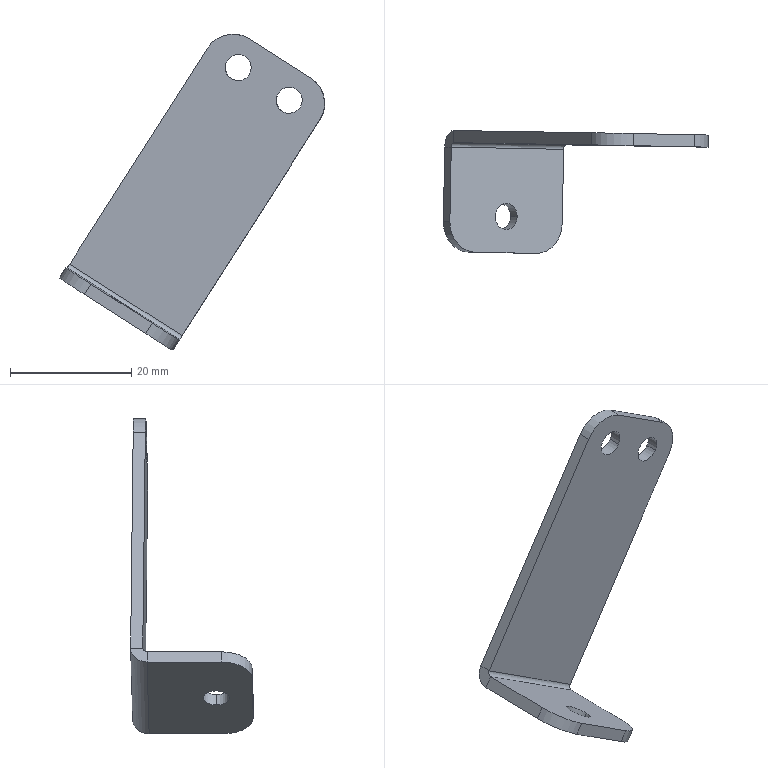Component | SolidWorks | DM17A08-02-003-1 | 1 solid | 24 faces | box 43.81 x 20.26 x 52.08 mm | volume 2829 mm3 | cylinder 12 | plane 12 | commonest cylinder face diameters 4.3 x6 10 x4 5.473 x1 1.473 x1
STEP:
#1=CARTESIAN_POINT('',(24.753,18.88,37.793));
#2=VERTEX_POINT('',#1);
#3=CARTESIAN_POINT('',(24.895,18.877,37.702));
#4=VERTEX_POINT('',#3);
#5=CARTESIAN_POINT('',(24.824,18.878,37.747));
#6=DIRECTION('',(-0.01873,-0.9998,0.));
#7=DIRECTION('',(0.843,-0.01579,-0.5377));
#8=AXIS2_PLACEMENT_3D('',#5,#6,#7);
#9=CIRCLE('',#8,0.08465);
#10=EDGE_CURVE('',#2,#4,#9,.T.);
#11=ORIENTED_EDGE('',*,*,#10,.F.);
#12=CARTESIAN_POINT('',(24.751,18.801,37.793));
#13=VERTEX_POINT('',#12);
#14=CARTESIAN_POINT('',(24.751,18.801,37.793));
#15=DIRECTION('',(-0.01873,-0.9998,0.));
#16=VECTOR('',#15,39.37);
#17=LINE('',#14,#16);
#18=EDGE_CURVE('',#2,#13,#17,.T.);
#19=ORIENTED_EDGE('',*,*,#18,.T.);
#20=CARTESIAN_POINT('',(24.894,18.798,37.702));
#21=VERTEX_POINT('',#20);
#22=CARTESIAN_POINT('',(24.823,18.8,37.747));
#23=DIRECTION('',(-0.01873,-0.9998,0.));
#24=DIRECTION('',(0.843,-0.01579,-0.5377));
#25=AXIS2_PLACEMENT_3D('',#22,#23,#24);
#26=CIRCLE('',#25,0.08465);
#27=EDGE_CURVE('',#13,#21,#26,.T.);
#28=ORIENTED_EDGE('',*,*,#27,.T.);
#29=CARTESIAN_POINT('',(24.894,18.798,37.702));
#30=DIRECTION('',(-0.01873,-0.9998,0.));
#31=VECTOR('',#30,39.37);
#32=LINE('',#29,#31);
#33=EDGE_CURVE('',#4,#21,#32,.T.);
#34=ORIENTED_EDGE('',*,*,#33,.F.);
#35=EDGE_LOOP('',(#11,#19,#28,#34));
#36=FACE_OUTER_BOUND('',#35,.T.);
#37=CARTESIAN_POINT('',(24.823,18.8,37.747));
#38=DIRECTION('',(-0.01873,-0.9998,0.));
#39=DIRECTION('',(0.843,-0.01579,-0.5377));
#40=AXIS2_PLACEMENT_3D('',#37,#38,#39);
#41=CYLINDRICAL_SURFACE('',#40,0.08465);
#42=ADVANCED_FACE('',(#36),#41,.F.);
#43=CARTESIAN_POINT('',(24.421,18.886,38.005));
#44=VERTEX_POINT('',#43);
#45=CARTESIAN_POINT('',(24.563,18.883,37.914));
#46=VERTEX_POINT('',#45);
#47=CARTESIAN_POINT('',(24.492,18.885,37.959));
#48=DIRECTION('',(-0.01873,-0.9998,0.));
#49=DIRECTION('',(0.843,-0.01579,-0.5377));
#50=AXIS2_PLACEMENT_3D('',#47,#48,#49);
#51=CIRCLE('',#50,0.08465);
#52=EDGE_CURVE('',#44,#46,#51,.T.);
#53=ORIENTED_EDGE('',*,*,#52,.F.);
#54=CARTESIAN_POINT('',(24.419,18.807,38.005));
#55=VERTEX_POINT('',#54);
#56=CARTESIAN_POINT('',(24.419,18.807,38.005));
#57=DIRECTION('',(-0.01873,-0.9998,0.));
#58=VECTOR('',#57,39.37);
#59=LINE('',#56,#58);
#60=EDGE_CURVE('',#44,#55,#59,.T.);
#61=ORIENTED_EDGE('',*,*,#60,.T.);
#62=CARTESIAN_POINT('',(24.562,18.805,37.914));
#63=VERTEX_POINT('',#62);
#64=CARTESIAN_POINT('',(24.491,18.806,37.959));
#65=DIRECTION('',(-0.01873,-0.9998,0.));
#66=DIRECTION('',(0.843,-0.01579,-0.5377));
#67=AXIS2_PLACEMENT_3D('',#64,#65,#66);
#68=CIRCLE('',#67,0.08465);
#69=EDGE_CURVE('',#55,#63,#68,.T.);
#70=ORIENTED_EDGE('',*,*,#69,.T.);
#71=CARTESIAN_POINT('',(24.562,18.805,37.914));
#72=DIRECTION('',(-0.01873,-0.9998,0.));
#73=VECTOR('',#72,39.37);
#74=LINE('',#71,#73);
#75=EDGE_CURVE('',#46,#63,#74,.T.);
#76=ORIENTED_EDGE('',*,*,#75,.F.);
#77=EDGE_LOOP('',(#53,#61,#70,#76));
#78=FACE_OUTER_BOUND('',#77,.T.);
#79=CARTESIAN_POINT('',(24.491,18.806,37.959));
#80=DIRECTION('',(-0.01873,-0.9998,0.));
#81=DIRECTION('',(0.843,-0.01579,-0.5377));
#82=AXIS2_PLACEMENT_3D('',#79,#80,#81);
#83=CYLINDRICAL_SURFACE('',#82,0.08465);
#84=ADVANCED_FACE('',(#78),#83,.F.);
#85=CARTESIAN_POINT('',(23.809,18.346,36.38));
#86=VERTEX_POINT('',#85);
#87=CARTESIAN_POINT('',(23.666,18.349,36.471));
#88=VERTEX_POINT('',#87);
#89=CARTESIAN_POINT('',(23.738,18.347,36.426));
#90=DIRECTION('',(-0.5377,0.01007,-0.8431));
#91=DIRECTION('',(0.01873,0.9998,0.));
#92=AXIS2_PLACEMENT_3D('',#89,#90,#91);
#93=CIRCLE('',#92,0.08465);
#94=EDGE_CURVE('',#86,#88,#93,.T.);
#95=ORIENTED_EDGE('',*,*,#94,.F.);
#96=CARTESIAN_POINT('',(23.767,18.347,36.314));
#97=VERTEX_POINT('',#96);
#98=CARTESIAN_POINT('',(23.767,18.347,36.314));
#99=DIRECTION('',(-0.5377,0.01007,-0.8431));
#100=VECTOR('',#99,39.37);
#101=LINE('',#98,#100);
#102=EDGE_CURVE('',#86,#97,#101,.T.);
#103=ORIENTED_EDGE('',*,*,#102,.T.);
#104=CARTESIAN_POINT('',(23.624,18.35,36.405));
#105=VERTEX_POINT('',#104);
#106=CARTESIAN_POINT('',(23.695,18.348,36.36));
#107=DIRECTION('',(-0.5377,0.01007,-0.8431));
#108=DIRECTION('',(-0.843,0.01579,0.5377));
#109=AXIS2_PLACEMENT_3D('',#106,#107,#108);
#110=CIRCLE('',#109,0.08465);
#111=EDGE_CURVE('',#97,#105,#110,.T.);
#112=ORIENTED_EDGE('',*,*,#111,.T.);
#113=CARTESIAN_POINT('',(23.624,18.35,36.405));
#114=DIRECTION('',(-0.5377,0.01007,-0.8431));
#115=VECTOR('',#114,39.37);
#116=LINE('',#113,#115);
#117=EDGE_CURVE('',#88,#105,#116,.T.);
#118=ORIENTED_EDGE('',*,*,#117,.F.);
#119=EDGE_LOOP('',(#95,#103,#112,#118));
#120=FACE_OUTER_BOUND('',#119,.T.);
#121=CARTESIAN_POINT('',(23.695,18.348,36.36));
#122=DIRECTION('',(-0.5377,0.01007,-0.8431));
#123=DIRECTION('',(-0.843,0.01579,0.5377));
#124=AXIS2_PLACEMENT_3D('',#121,#122,#123);
#125=CYLINDRICAL_SURFACE('',#124,0.08465);
#126=ADVANCED_FACE('',(#120),#125,.F.);
#127=CARTESIAN_POINT('',(24.069,18.785,36.127));
#128=VERTEX_POINT('',#127);
#129=CARTESIAN_POINT('',(24.111,18.784,36.193));
#130=VERTEX_POINT('',#129);
#131=CARTESIAN_POINT('',(24.069,18.785,36.127));
#132=DIRECTION('',(0.5377,-0.01007,0.8431));
#133=VECTOR('',#132,39.37);
#134=LINE('',#131,#133);
#135=EDGE_CURVE('',#128,#130,#134,.T.);
#136=ORIENTED_EDGE('',*,*,#135,.F.);
#137=CARTESIAN_POINT('',(24.129,18.891,36.217));
#138=VERTEX_POINT('',#137);
#139=CARTESIAN_POINT('',(24.126,18.784,36.217));
#140=DIRECTION('',(-0.843,0.01579,0.5377));
#141=DIRECTION('',(0.01873,0.9998,0.));
#142=AXIS2_PLACEMENT_3D('',#139,#140,#141);
#143=CIRCLE('',#142,0.1077);
#144=EDGE_CURVE('',#138,#128,#143,.T.);
#145=ORIENTED_EDGE('',*,*,#144,.F.);
#146=CARTESIAN_POINT('',(24.127,18.813,36.217));
#147=VERTEX_POINT('',#146);
#148=CARTESIAN_POINT('',(24.127,18.813,36.217));
#149=DIRECTION('',(0.01873,0.9998,-0.));
#150=VECTOR('',#149,39.37);
#151=LINE('',#148,#150);
#152=EDGE_CURVE('',#147,#138,#151,.T.);
#153=ORIENTED_EDGE('',*,*,#152,.F.);
#154=CARTESIAN_POINT('',(24.126,18.784,36.217));
#155=DIRECTION('',(-0.843,0.01579,0.5377));
#156=DIRECTION('',(0.01873,0.9998,0.));
#157=AXIS2_PLACEMENT_3D('',#154,#155,#156);
#158=CIRCLE('',#157,0.029);
#159=EDGE_CURVE('',#147,#130,#158,.T.);
#160=ORIENTED_EDGE('',*,*,#159,.T.);
#161=EDGE_LOOP('',(#136,#145,#153,#160));
#162=FACE_OUTER_BOUND('',#161,.T.);
#163=CARTESIAN_POINT('',(24.069,18.785,36.127));
#164=DIRECTION('',(0.843,-0.01579,-0.5377));
#165=DIRECTION('',(0.01873,0.9998,-0.));
#166=AXIS2_PLACEMENT_3D('',#163,#164,#165);
#167=PLANE('',#166);
#168=ADVANCED_FACE('',(#162),#167,.T.);
#169=CARTESIAN_POINT('',(24.102,18.301,36.193));
#170=VERTEX_POINT('',#169);
#171=CARTESIAN_POINT('',(24.113,18.892,36.193));
#172=DIRECTION('',(-0.01873,-0.9998,0.));
#173=VECTOR('',#172,39.37);
#174=LINE('',#171,#173);
#175=EDGE_CURVE('',#130,#170,#174,.T.);
#176=ORIENTED_EDGE('',*,*,#175,.T.);
#177=CARTESIAN_POINT('',(24.06,18.302,36.127));
#178=VERTEX_POINT('',#177);
#179=CARTESIAN_POINT('',(24.117,18.301,36.217));
#180=DIRECTION('',(-0.5377,0.01007,-0.8431));
#181=VECTOR('',#180,39.37);
#182=LINE('',#179,#181);
#183=EDGE_CURVE('',#170,#178,#182,.T.);
#184=ORIENTED_EDGE('',*,*,#183,.T.);
#185=CARTESIAN_POINT('',(24.071,18.892,36.127));
#186=DIRECTION('',(-0.01873,-0.9998,0.));
#187=VECTOR('',#186,39.37);
#188=LINE('',#185,#187);
#189=EDGE_CURVE('',#128,#178,#188,.T.);
#190=ORIENTED_EDGE('',*,*,#189,.F.);
#191=ORIENTED_EDGE('',*,*,#135,.T.);
#192=EDGE_LOOP('',(#176,#184,#190,#191));
#193=FACE_OUTER_BOUND('',#192,.T.);
#194=CARTESIAN_POINT('',(24.127,18.813,36.217));
#195=DIRECTION('',(0.843,-0.01579,-0.5377));
#196=DIRECTION('',(0.01873,0.9998,-0.));
#197=AXIS2_PLACEMENT_3D('',#194,#195,#196);
#198=PLANE('',#197);
#199=ADVANCED_FACE('',(#193),#198,.T.);
#200=CARTESIAN_POINT('',(23.398,18.905,36.683));
#201=VERTEX_POINT('',#200);
#202=CARTESIAN_POINT('',(23.397,18.826,36.683));
#203=VERTEX_POINT('',#202);
#204=CARTESIAN_POINT('',(23.398,18.905,36.683));
#205=DIRECTION('',(-0.01873,-0.9998,0.));
#206=VECTOR('',#205,39.37);
#207=LINE('',#204,#206);
#208=EDGE_CURVE('',#201,#203,#207,.T.);
#209=ORIENTED_EDGE('',*,*,#208,.F.);
#210=CARTESIAN_POINT('',(23.338,18.798,36.592));
#211=VERTEX_POINT('',#210);
#212=CARTESIAN_POINT('',(23.396,18.797,36.683));
#213=DIRECTION('',(-0.843,0.01579,0.5377));
#214=DIRECTION('',(0.01873,0.9998,0.));
#215=AXIS2_PLACEMENT_3D('',#212,#213,#214);
#216=CIRCLE('',#215,0.1077);
#217=EDGE_CURVE('',#201,#211,#216,.T.);
#218=ORIENTED_EDGE('',*,*,#217,.T.);
#219=CARTESIAN_POINT('',(23.381,18.798,36.659));
#220=VERTEX_POINT('',#219);
#221=CARTESIAN_POINT('',(23.381,18.798,36.659));
#222=DIRECTION('',(-0.5377,0.01007,-0.8431));
#223=VECTOR('',#222,39.37);
#224=LINE('',#221,#223);
#225=EDGE_CURVE('',#220,#211,#224,.T.);
#226=ORIENTED_EDGE('',*,*,#225,.F.);
#227=CARTESIAN_POINT('',(23.396,18.797,36.683));
#228=DIRECTION('',(-0.843,0.01579,0.5377));
#229=DIRECTION('',(0.01873,0.9998,0.));
#230=AXIS2_PLACEMENT_3D('',#227,#228,#229);
#231=CIRCLE('',#230,0.029);
#232=EDGE_CURVE('',#203,#220,#231,.T.);
#233=ORIENTED_EDGE('',*,*,#232,.F.);
#234=EDGE_LOOP('',(#209,#218,#226,#233));
#235=FACE_OUTER_BOUND('',#234,.T.);
#236=CARTESIAN_POINT('',(23.398,18.905,36.683));
#237=DIRECTION('',(-0.843,0.01579,0.5377));
#238=DIRECTION('',(-0.01873,-0.9998,0.));
#239=AXIS2_PLACEMENT_3D('',#236,#237,#238);
#240=PLANE('',#239);
#241=ADVANCED_FACE('',(#235),#240,.T.);
#242=CARTESIAN_POINT('',(24.292,18.81,38.086));
#243=VERTEX_POINT('',#242);
#244=CARTESIAN_POINT('',(24.397,18.808,38.252));
#245=DIRECTION('',(-0.5377,0.01007,-0.8431));
#246=VECTOR('',#245,39.37);
#247=LINE('',#244,#246);
#248=EDGE_CURVE('',#243,#203,#247,.T.);
#249=ORIENTED_EDGE('',*,*,#248,.F.);
#250=CARTESIAN_POINT('',(24.293,18.888,38.086));
#251=VERTEX_POINT('',#250);
#252=CARTESIAN_POINT('',(24.291,18.781,38.086));
#253=DIRECTION('',(0.01873,0.9998,-0.));
#254=VECTOR('',#253,39.37);
#255=LINE('',#252,#254);
#256=EDGE_CURVE('',#243,#251,#255,.T.);
#257=ORIENTED_EDGE('',*,*,#256,.T.);
#258=CARTESIAN_POINT('',(24.399,18.886,38.252));
#259=DIRECTION('',(-0.5377,0.01007,-0.8431));
#260=VECTOR('',#259,39.37);
#261=LINE('',#258,#260);
#262=EDGE_CURVE('',#251,#201,#261,.T.);
#263=ORIENTED_EDGE('',*,*,#262,.T.);
#264=ORIENTED_EDGE('',*,*,#208,.T.);
#265=EDGE_LOOP('',(#249,#257,#263,#264));
#266=FACE_OUTER_BOUND('',#265,.T.);
#267=CARTESIAN_POINT('',(23.381,18.798,36.659));
#268=DIRECTION('',(-0.843,0.01579,0.5377));
#269=DIRECTION('',(-0.01873,-0.9998,0.));
#270=AXIS2_PLACEMENT_3D('',#267,#268,#269);
#271=PLANE('',#270);
#272=ADVANCED_FACE('',(#266),#271,.T.);
#273=CARTESIAN_POINT('',(23.738,18.347,36.426));
#274=DIRECTION('',(-0.5377,0.01007,-0.8431));
#275=DIRECTION('',(0.01873,0.9998,0.));
#276=AXIS2_PLACEMENT_3D('',#273,#274,#275);
#277=CIRCLE('',#276,0.08465);
#278=EDGE_CURVE('',#88,#86,#277,.T.);
#279=ORIENTED_EDGE('',*,*,#278,.T.);
#280=ORIENTED_EDGE('',*,*,#94,.T.);
#281=EDGE_LOOP('',(#279,#280));
#282=FACE_BOUND('',#281,.T.);
#283=CARTESIAN_POINT('',(23.932,18.108,36.299));
#284=VERTEX_POINT('',#283);
#285=CARTESIAN_POINT('',(23.534,18.115,36.553));
#286=VERTEX_POINT('',#285);
#287=CARTESIAN_POINT('',(24.098,18.104,36.193));
#288=DIRECTION('',(-0.843,0.01579,0.5377));
#289=VECTOR('',#288,39.37);
#290=LINE('',#287,#289);
#291=EDGE_CURVE('',#284,#286,#290,.T.);
#292=ORIENTED_EDGE('',*,*,#291,.F.);
#293=CARTESIAN_POINT('',(23.936,18.304,36.299));
#294=DIRECTION('',(0.5377,-0.01007,0.8431));
#295=DIRECTION('',(0.01873,0.9998,0.));
#296=AXIS2_PLACEMENT_3D('',#293,#294,#295);
#297=CIRCLE('',#296,0.1969);
#298=EDGE_CURVE('',#284,#170,#297,.T.);
#299=ORIENTED_EDGE('',*,*,#298,.T.);
#300=ORIENTED_EDGE('',*,*,#175,.F.);
#301=CARTESIAN_POINT('',(24.111,18.784,36.193));
#302=DIRECTION('',(-0.843,0.01579,0.5377));
#303=VECTOR('',#302,39.37);
#304=LINE('',#301,#303);
#305=EDGE_CURVE('',#130,#220,#304,.T.);
#306=ORIENTED_EDGE('',*,*,#305,.T.);
#307=CARTESIAN_POINT('',(23.372,18.315,36.659));
#308=VERTEX_POINT('',#307);
#309=CARTESIAN_POINT('',(23.383,18.905,36.659));
#310=DIRECTION('',(-0.01873,-0.9998,0.));
#311=VECTOR('',#310,39.37);
#312=LINE('',#309,#311);
#313=EDGE_CURVE('',#220,#308,#312,.T.);
#314=ORIENTED_EDGE('',*,*,#313,.T.);
#315=CARTESIAN_POINT('',(23.538,18.312,36.553));
#316=DIRECTION('',(0.5377,-0.01007,0.8431));
#317=DIRECTION('',(0.01873,0.9998,0.));
#318=AXIS2_PLACEMENT_3D('',#315,#316,#317);
#319=CIRCLE('',#318,0.1969);
#320=EDGE_CURVE('',#308,#286,#319,.T.);
#321=ORIENTED_EDGE('',*,*,#320,.T.);
#322=EDGE_LOOP('',(#292,#299,#300,#306,#314,#321));
#323=FACE_OUTER_BOUND('',#322,.T.);
#324=CARTESIAN_POINT('',(24.113,18.892,36.193));
#325=DIRECTION('',(-0.5377,0.01007,-0.8431));
#326=DIRECTION('',(0.01873,0.9998,-0.));
#327=AXIS2_PLACEMENT_3D('',#324,#325,#326);
#328=PLANE('',#327);
#329=ADVANCED_FACE('',(#282,#323),#328,.F.);
#330=CARTESIAN_POINT('',(23.89,18.108,36.233));
#331=VERTEX_POINT('',#330);
#332=CARTESIAN_POINT('',(23.492,18.116,36.487));
#333=VERTEX_POINT('',#332);
#334=CARTESIAN_POINT('',(24.056,18.105,36.127));
#335=DIRECTION('',(-0.843,0.01579,0.5377));
#336=VECTOR('',#335,39.37);
#337=LINE('',#334,#336);
#338=EDGE_CURVE('',#331,#333,#337,.T.);
#339=ORIENTED_EDGE('',*,*,#338,.F.);
#340=CARTESIAN_POINT('',(23.89,18.108,36.233));
#341=DIRECTION('',(0.5377,-0.01007,0.8431));
#342=VECTOR('',#341,39.37);
#343=LINE('',#340,#342);
#344=EDGE_CURVE('',#331,#284,#343,.T.);
#345=ORIENTED_EDGE('',*,*,#344,.T.);
#346=ORIENTED_EDGE('',*,*,#291,.T.);
#347=CARTESIAN_POINT('',(23.492,18.116,36.487));
#348=DIRECTION('',(-0.5377,0.01007,-0.8431));
#349=VECTOR('',#348,39.37);
#350=LINE('',#347,#349);
#351=EDGE_CURVE('',#286,#333,#350,.T.);
#352=ORIENTED_EDGE('',*,*,#351,.T.);
#353=EDGE_LOOP('',(#339,#345,#346,#352));
#354=FACE_OUTER_BOUND('',#353,.T.);
#355=CARTESIAN_POINT('',(24.056,18.105,36.127));
#356=DIRECTION('',(-0.01873,-0.9998,0.));
#357=DIRECTION('',(0.843,-0.01579,-0.5377));
#358=AXIS2_PLACEMENT_3D('',#355,#356,#357);
#359=PLANE('',#358);
#360=ADVANCED_FACE('',(#354),#359,.T.);
#361=CARTESIAN_POINT('',(23.695,18.348,36.36));
#362=DIRECTION('',(-0.5377,0.01007,-0.8431));
#363=DIRECTION('',(-0.843,0.01579,0.5377));
#364=AXIS2_PLACEMENT_3D('',#361,#362,#363);
#365=CIRCLE('',#364,0.08465);
#366=EDGE_CURVE('',#105,#97,#365,.T.);
#367=ORIENTED_EDGE('',*,*,#366,.F.);
#368=ORIENTED_EDGE('',*,*,#111,.F.);
#369=EDGE_LOOP('',(#367,#368));
#370=FACE_BOUND('',#369,.T.);
#371=ORIENTED_EDGE('',*,*,#189,.T.);
#372=CARTESIAN_POINT('',(23.894,18.305,36.233));
#373=DIRECTION('',(-0.5377,0.01007,-0.8431));
#374=DIRECTION('',(0.01873,0.9998,0.));
#375=AXIS2_PLACEMENT_3D('',#372,#373,#374);
#376=CIRCLE('',#375,0.1969);
#377=EDGE_CURVE('',#178,#331,#376,.T.);
#378=ORIENTED_EDGE('',*,*,#377,.T.);
#379=ORIENTED_EDGE('',*,*,#338,.T.);
#380=CARTESIAN_POINT('',(23.329,18.316,36.592));
#381=VERTEX_POINT('',#380);
#382=CARTESIAN_POINT('',(23.495,18.313,36.487));
#383=DIRECTION('',(-0.5377,0.01007,-0.8431));
#384=DIRECTION('',(0.01873,0.9998,0.));
#385=AXIS2_PLACEMENT_3D('',#382,#383,#384);
#386=CIRCLE('',#385,0.1969);
#387=EDGE_CURVE('',#333,#381,#386,.T.);
#388=ORIENTED_EDGE('',*,*,#387,.T.);
#389=CARTESIAN_POINT('',(23.34,18.906,36.592));
#390=DIRECTION('',(-0.01873,-0.9998,0.));
#391=VECTOR('',#390,39.37);
#392=LINE('',#389,#391);
#393=EDGE_CURVE('',#211,#381,#392,.T.);
#394=ORIENTED_EDGE('',*,*,#393,.F.);
#395=CARTESIAN_POINT('',(24.069,18.785,36.127));
#396=DIRECTION('',(-0.843,0.01579,0.5377));
#397=VECTOR('',#396,39.37);
#398=LINE('',#395,#397);
#399=EDGE_CURVE('',#128,#211,#398,.T.);
#400=ORIENTED_EDGE('',*,*,#399,.F.);
#401=EDGE_LOOP('',(#371,#378,#379,#388,#394,#400));
#402=FACE_OUTER_BOUND('',#401,.T.);
#403=CARTESIAN_POINT('',(24.071,18.892,36.127));
#404=DIRECTION('',(-0.5377,0.01007,-0.8431));
#405=DIRECTION('',(0.01873,0.9998,-0.));
#406=AXIS2_PLACEMENT_3D('',#403,#404,#405);
#407=PLANE('',#406);
#408=ADVANCED_FACE('',(#370,#402),#407,.T.);
#409=ORIENTED_EDGE('',*,*,#217,.F.);
#410=CARTESIAN_POINT('',(24.129,18.891,36.217));
#411=DIRECTION('',(-0.843,0.01579,0.5377));
#412=VECTOR('',#411,39.37);
#413=LINE('',#410,#412);
#414=EDGE_CURVE('',#138,#201,#413,.T.);
#415=ORIENTED_EDGE('',*,*,#414,.F.);
#416=ORIENTED_EDGE('',*,*,#144,.T.);
#417=ORIENTED_EDGE('',*,*,#399,.T.);
#418=EDGE_LOOP('',(#409,#415,#416,#417));
#419=FACE_OUTER_BOUND('',#418,.T.);
#420=CARTESIAN_POINT('',(24.126,18.784,36.217));
#421=DIRECTION('',(-0.843,0.01579,0.5377));
#422=DIRECTION('',(-0.01873,-0.9998,0.));
#423=AXIS2_PLACEMENT_3D('',#420,#421,#422);
#424=CYLINDRICAL_SURFACE('',#423,0.1077);
#425=ADVANCED_FACE('',(#419),#424,.T.);
#426=CARTESIAN_POINT('',(24.824,18.878,37.747));
#427=DIRECTION('',(-0.01873,-0.9998,0.));
#428=DIRECTION('',(0.843,-0.01579,-0.5377));
#429=AXIS2_PLACEMENT_3D('',#426,#427,#428);
#430=CIRCLE('',#429,0.08465);
#431=EDGE_CURVE('',#4,#2,#430,.T.);
#432=ORIENTED_EDGE('',*,*,#431,.T.);
#433=ORIENTED_EDGE('',*,*,#10,.T.);
#434=EDGE_LOOP('',(#432,#433));
#435=FACE_BOUND('',#434,.T.);
#436=CARTESIAN_POINT('',(24.492,18.885,37.959));
#437=DIRECTION('',(-0.01873,-0.9998,0.));
#438=DIRECTION('',(0.843,-0.01579,-0.5377));
#439=AXIS2_PLACEMENT_3D('',#436,#437,#438);
#440=CIRCLE('',#439,0.08465);
#441=EDGE_CURVE('',#46,#44,#440,.T.);
#442=ORIENTED_EDGE('',*,*,#441,.T.);
#443=ORIENTED_EDGE('',*,*,#52,.T.);
#444=EDGE_LOOP('',(#442,#443));
#445=FACE_BOUND('',#444,.T.);
#446=CARTESIAN_POINT('',(24.963,18.876,37.892));
#447=VERTEX_POINT('',#446);
#448=CARTESIAN_POINT('',(24.565,18.883,38.146));
#449=VERTEX_POINT('',#448);
#450=CARTESIAN_POINT('',(25.129,18.873,37.786));
#451=DIRECTION('',(-0.843,0.01579,0.5377));
#452=VECTOR('',#451,39.37);
#453=LINE('',#450,#452);
#454=EDGE_CURVE('',#447,#449,#453,.T.);
#455=ORIENTED_EDGE('',*,*,#454,.F.);
#456=CARTESIAN_POINT('',(25.023,18.875,37.62));
#457=VERTEX_POINT('',#456);
#458=CARTESIAN_POINT('',(24.857,18.878,37.726));
#459=DIRECTION('',(0.01873,0.9998,-0.));
#460=DIRECTION('',(-0.843,0.01579,0.5377));
#461=AXIS2_PLACEMENT_3D('',#458,#459,#460);
#462=CIRCLE('',#461,0.1969);
#463=EDGE_CURVE('',#447,#457,#462,.T.);
#464=ORIENTED_EDGE('',*,*,#463,.T.);
#465=CARTESIAN_POINT('',(25.129,18.873,37.786));
#466=DIRECTION('',(-0.5377,0.01007,-0.8431));
#467=VECTOR('',#466,39.37);
#468=LINE('',#465,#467);
#469=EDGE_CURVE('',#457,#138,#468,.T.);
#470=ORIENTED_EDGE('',*,*,#469,.T.);
#471=ORIENTED_EDGE('',*,*,#414,.T.);
#472=ORIENTED_EDGE('',*,*,#262,.F.);
#473=CARTESIAN_POINT('',(24.459,18.885,37.98));
#474=DIRECTION('',(0.01873,0.9998,-0.));
#475=DIRECTION('',(-0.843,0.01579,0.5377));
#476=AXIS2_PLACEMENT_3D('',#473,#474,#475);
#477=CIRCLE('',#476,0.1969);
#478=EDGE_CURVE('',#251,#449,#477,.T.);
#479=ORIENTED_EDGE('',*,*,#478,.T.);
#480=EDGE_LOOP('',(#455,#464,#470,#471,#472,#479));
#481=FACE_OUTER_BOUND('',#480,.T.);
#482=CARTESIAN_POINT('',(25.129,18.873,37.786));
#483=DIRECTION('',(0.01873,0.9998,-0.));
#484=DIRECTION('',(-0.843,0.01579,0.5377));
#485=AXIS2_PLACEMENT_3D('',#482,#483,#484);
#486=PLANE('',#485);
#487=ADVANCED_FACE('',(#435,#445,#481),#486,.T.);
#488=CARTESIAN_POINT('',(24.962,18.797,37.892));
#489=VERTEX_POINT('',#488);
#490=CARTESIAN_POINT('',(24.563,18.804,38.146));
#491=VERTEX_POINT('',#490);
#492=CARTESIAN_POINT('',(25.127,18.794,37.786));
#493=DIRECTION('',(-0.843,0.01579,0.5377));
#494=VECTOR('',#493,39.37);
#495=LINE('',#492,#494);
#496=EDGE_CURVE('',#489,#491,#495,.T.);
#497=ORIENTED_EDGE('',*,*,#496,.F.);
#498=CARTESIAN_POINT('',(24.962,18.797,37.892));
#499=DIRECTION('',(0.01873,0.9998,-0.));
#500=VECTOR('',#499,39.37);
#501=LINE('',#498,#500);
#502=EDGE_CURVE('',#489,#447,#501,.T.);
#503=ORIENTED_EDGE('',*,*,#502,.T.);
#504=ORIENTED_EDGE('',*,*,#454,.T.);
#505=CARTESIAN_POINT('',(24.563,18.804,38.146));
#506=DIRECTION('',(-0.01873,-0.9998,0.));
#507=VECTOR('',#506,39.37);
#508=LINE('',#505,#507);
#509=EDGE_CURVE('',#449,#491,#508,.T.);
#510=ORIENTED_EDGE('',*,*,#509,.T.);
#511=EDGE_LOOP('',(#497,#503,#504,#510));
#512=FACE_OUTER_BOUND('',#511,.T.);
#513=CARTESIAN_POINT('',(25.127,18.794,37.786));
#514=DIRECTION('',(0.5377,-0.01007,0.8431));
#515=DIRECTION('',(0.843,-0.01579,-0.5377));
#516=AXIS2_PLACEMENT_3D('',#513,#514,#515);
#517=PLANE('',#516);
#518=ADVANCED_FACE('',(#512),#517,.T.);
#519=CARTESIAN_POINT('',(24.823,18.8,37.747));
#520=DIRECTION('',(-0.01873,-0.9998,0.));
#521=DIRECTION('',(0.843,-0.01579,-0.5377));
#522=AXIS2_PLACEMENT_3D('',#519,#520,#521);
#523=CIRCLE('',#522,0.08465);
#524=EDGE_CURVE('',#21,#13,#523,.T.);
#525=ORIENTED_EDGE('',*,*,#524,.F.);
#526=ORIENTED_EDGE('',*,*,#27,.F.);
#527=EDGE_LOOP('',(#525,#526));
#528=FACE_BOUND('',#527,.T.);
#529=CARTESIAN_POINT('',(24.491,18.806,37.959));
#530=DIRECTION('',(-0.01873,-0.9998,0.));
#531=DIRECTION('',(0.843,-0.01579,-0.5377));
#532=AXIS2_PLACEMENT_3D('',#529,#530,#531);
#533=CIRCLE('',#532,0.08465);
#534=EDGE_CURVE('',#63,#55,#533,.T.);
#535=ORIENTED_EDGE('',*,*,#534,.F.);
#536=ORIENTED_EDGE('',*,*,#69,.F.);
#537=EDGE_LOOP('',(#535,#536));
#538=FACE_BOUND('',#537,.T.);
#539=CARTESIAN_POINT('',(25.022,18.796,37.62));
#540=VERTEX_POINT('',#539);
#541=CARTESIAN_POINT('',(25.127,18.794,37.786));
#542=DIRECTION('',(-0.5377,0.01007,-0.8431));
#543=VECTOR('',#542,39.37);
#544=LINE('',#541,#543);
#545=EDGE_CURVE('',#540,#147,#544,.T.);
#546=ORIENTED_EDGE('',*,*,#545,.F.);
#547=CARTESIAN_POINT('',(24.856,18.799,37.726));
#548=DIRECTION('',(-0.01873,-0.9998,0.));
#549=DIRECTION('',(-0.843,0.01579,0.5377));
#550=AXIS2_PLACEMENT_3D('',#547,#548,#549);
#551=CIRCLE('',#550,0.1969);
#552=EDGE_CURVE('',#540,#489,#551,.T.);
#553=ORIENTED_EDGE('',*,*,#552,.T.);
#554=ORIENTED_EDGE('',*,*,#496,.T.);
#555=CARTESIAN_POINT('',(24.457,18.806,37.98));
#556=DIRECTION('',(-0.01873,-0.9998,0.));
#557=DIRECTION('',(-0.843,0.01579,0.5377));
#558=AXIS2_PLACEMENT_3D('',#555,#556,#557);
#559=CIRCLE('',#558,0.1969);
#560=EDGE_CURVE('',#491,#243,#559,.T.);
#561=ORIENTED_EDGE('',*,*,#560,.T.);
#562=ORIENTED_EDGE('',*,*,#248,.T.);
#563=CARTESIAN_POINT('',(24.127,18.813,36.217));
#564=DIRECTION('',(-0.843,0.01579,0.5377));
#565=VECTOR('',#564,39.37);
#566=LINE('',#563,#565);
#567=EDGE_CURVE('',#147,#203,#566,.T.);
#568=ORIENTED_EDGE('',*,*,#567,.F.);
#569=EDGE_LOOP('',(#546,#553,#554,#561,#562,#568));
#570=FACE_OUTER_BOUND('',#569,.T.);
#571=CARTESIAN_POINT('',(25.127,18.794,37.786));
#572=DIRECTION('',(0.01873,0.9998,-0.));
#573=DIRECTION('',(-0.843,0.01579,0.5377));
#574=AXIS2_PLACEMENT_3D('',#571,#572,#573);
#575=PLANE('',#574);
#576=ADVANCED_FACE('',(#528,#538,#570),#575,.F.);
#577=ORIENTED_EDGE('',*,*,#232,.T.);
#578=ORIENTED_EDGE('',*,*,#305,.F.);
#579=ORIENTED_EDGE('',*,*,#159,.F.);
#580=ORIENTED_EDGE('',*,*,#567,.T.);
#581=EDGE_LOOP('',(#577,#578,#579,#580));
#582=FACE_OUTER_BOUND('',#581,.T.);
#583=CARTESIAN_POINT('',(24.126,18.784,36.217));
#584=DIRECTION('',(-0.843,0.01579,0.5377));
#585=DIRECTION('',(-0.01873,-0.9998,0.));
#586=AXIS2_PLACEMENT_3D('',#583,#584,#585);
#587=CYLINDRICAL_SURFACE('',#586,0.029);
#588=ADVANCED_FACE('',(#582),#587,.F.);
#589=ORIENTED_EDGE('',*,*,#469,.F.);
#590=CARTESIAN_POINT('',(25.021,18.767,37.62));
#591=DIRECTION('',(-0.01873,-0.9998,0.));
#592=VECTOR('',#591,39.37);
#593=LINE('',#590,#592);
#594=EDGE_CURVE('',#457,#540,#593,.T.);
#595=ORIENTED_EDGE('',*,*,#594,.T.);
#596=ORIENTED_EDGE('',*,*,#545,.T.);
#597=ORIENTED_EDGE('',*,*,#152,.T.);
#598=EDGE_LOOP('',(#589,#595,#596,#597));
#599=FACE_OUTER_BOUND('',#598,.T.);
#600=CARTESIAN_POINT('',(24.126,18.784,36.217));
#601=DIRECTION('',(0.843,-0.01579,-0.5377));
#602=DIRECTION('',(0.01873,0.9998,-0.));
#603=AXIS2_PLACEMENT_3D('',#600,#601,#602);
#604=PLANE('',#603);
#605=ADVANCED_FACE('',(#599),#604,.T.);
#606=ORIENTED_EDGE('',*,*,#393,.T.);
#607=CARTESIAN_POINT('',(23.372,18.315,36.659));
#608=DIRECTION('',(0.5377,-0.01007,0.8431));
#609=VECTOR('',#608,39.37);
#610=LINE('',#607,#609);
#611=EDGE_CURVE('',#381,#308,#610,.T.);
#612=ORIENTED_EDGE('',*,*,#611,.T.);
#613=ORIENTED_EDGE('',*,*,#313,.F.);
#614=ORIENTED_EDGE('',*,*,#225,.T.);
#615=EDGE_LOOP('',(#606,#612,#613,#614));
#616=FACE_OUTER_BOUND('',#615,.T.);
#617=CARTESIAN_POINT('',(23.396,18.797,36.683));
#618=DIRECTION('',(0.843,-0.01579,-0.5377));
#619=DIRECTION('',(0.01873,0.9998,-0.));
#620=AXIS2_PLACEMENT_3D('',#617,#618,#619);
#621=PLANE('',#620);
#622=ADVANCED_FACE('',(#616),#621,.F.);
#623=ORIENTED_EDGE('',*,*,#102,.F.);
#624=ORIENTED_EDGE('',*,*,#278,.F.);
#625=ORIENTED_EDGE('',*,*,#117,.T.);
#626=ORIENTED_EDGE('',*,*,#366,.T.);
#627=EDGE_LOOP('',(#623,#624,#625,#626));
#628=FACE_OUTER_BOUND('',#627,.T.);
#629=CARTESIAN_POINT('',(23.695,18.348,36.36));
#630=DIRECTION('',(-0.5377,0.01007,-0.8431));
#631=DIRECTION('',(-0.843,0.01579,0.5377));
#632=AXIS2_PLACEMENT_3D('',#629,#630,#631);
#633=CYLINDRICAL_SURFACE('',#632,0.08465);
#634=ADVANCED_FACE('',(#628),#633,.F.);
#635=ORIENTED_EDGE('',*,*,#60,.F.);
#636=ORIENTED_EDGE('',*,*,#441,.F.);
#637=ORIENTED_EDGE('',*,*,#75,.T.);
#638=ORIENTED_EDGE('',*,*,#534,.T.);
#639=EDGE_LOOP('',(#635,#636,#637,#638));
#640=FACE_OUTER_BOUND('',#639,.T.);
#641=CARTESIAN_POINT('',(24.491,18.806,37.959));
#642=DIRECTION('',(-0.01873,-0.9998,0.));
#643=DIRECTION('',(0.843,-0.01579,-0.5377));
#644=AXIS2_PLACEMENT_3D('',#641,#642,#643);
#645=CYLINDRICAL_SURFACE('',#644,0.08465);
#646=ADVANCED_FACE('',(#640),#645,.F.);
#647=ORIENTED_EDGE('',*,*,#18,.F.);
#648=ORIENTED_EDGE('',*,*,#431,.F.);
#649=ORIENTED_EDGE('',*,*,#33,.T.);
#650=ORIENTED_EDGE('',*,*,#524,.T.);
#651=EDGE_LOOP('',(#647,#648,#649,#650));
#652=FACE_OUTER_BOUND('',#651,.T.);
#653=CARTESIAN_POINT('',(24.823,18.8,37.747));
#654=DIRECTION('',(-0.01873,-0.9998,0.));
#655=DIRECTION('',(0.843,-0.01579,-0.5377));
#656=AXIS2_PLACEMENT_3D('',#653,#654,#655);
#657=CYLINDRICAL_SURFACE('',#656,0.08465);
#658=ADVANCED_FACE('',(#652),#657,.F.);
#659=ORIENTED_EDGE('',*,*,#552,.F.);
#660=ORIENTED_EDGE('',*,*,#594,.F.);
#661=ORIENTED_EDGE('',*,*,#463,.F.);
#662=ORIENTED_EDGE('',*,*,#502,.F.);
#663=EDGE_LOOP('',(#659,#660,#661,#662));
#664=FACE_OUTER_BOUND('',#663,.T.);
#665=CARTESIAN_POINT('',(24.856,18.799,37.726));
#666=DIRECTION('',(0.01873,0.9998,-0.));
#667=DIRECTION('',(-0.843,0.01579,0.5377));
#668=AXIS2_PLACEMENT_3D('',#665,#666,#667);
#669=CYLINDRICAL_SURFACE('',#668,0.1969);
#670=ADVANCED_FACE('',(#664),#669,.T.);
#671=ORIENTED_EDGE('',*,*,#560,.F.);
#672=ORIENTED_EDGE('',*,*,#509,.F.);
#673=ORIENTED_EDGE('',*,*,#478,.F.);
#674=ORIENTED_EDGE('',*,*,#256,.F.);
#675=EDGE_LOOP('',(#671,#672,#673,#674));
#676=FACE_OUTER_BOUND('',#675,.T.);
#677=CARTESIAN_POINT('',(24.457,18.777,37.98));
#678=DIRECTION('',(0.01873,0.9998,-0.));
#679=DIRECTION('',(-0.843,0.01579,0.5377));
#680=AXIS2_PLACEMENT_3D('',#677,#678,#679);
#681=CYLINDRICAL_SURFACE('',#680,0.1969);
#682=ADVANCED_FACE('',(#676),#681,.T.);
#683=ORIENTED_EDGE('',*,*,#377,.F.);
#684=ORIENTED_EDGE('',*,*,#183,.F.);
#685=ORIENTED_EDGE('',*,*,#298,.F.);
#686=ORIENTED_EDGE('',*,*,#344,.F.);
#687=EDGE_LOOP('',(#683,#684,#685,#686));
#688=FACE_OUTER_BOUND('',#687,.T.);
#689=CARTESIAN_POINT('',(23.894,18.305,36.233));
#690=DIRECTION('',(0.5377,-0.01007,0.8431));
#691=DIRECTION('',(0.843,-0.01579,-0.5377));
#692=AXIS2_PLACEMENT_3D('',#689,#690,#691);
#693=CYLINDRICAL_SURFACE('',#692,0.1969);
#694=ADVANCED_FACE('',(#688),#693,.T.);
#695=ORIENTED_EDGE('',*,*,#387,.F.);
#696=ORIENTED_EDGE('',*,*,#351,.F.);
#697=ORIENTED_EDGE('',*,*,#320,.F.);
#698=ORIENTED_EDGE('',*,*,#611,.F.);
#699=EDGE_LOOP('',(#695,#696,#697,#698));
#700=FACE_OUTER_BOUND('',#699,.T.);
#701=CARTESIAN_POINT('',(23.553,18.312,36.577));
#702=DIRECTION('',(-0.5377,0.01007,-0.8431));
#703=DIRECTION('',(-0.843,0.01579,0.5377));
#704=AXIS2_PLACEMENT_3D('',#701,#702,#703);
#705=CYLINDRICAL_SURFACE('',#704,0.1969);
#706=ADVANCED_FACE('',(#700),#705,.T.);
#707=CLOSED_SHELL('',(#42,#84,#126,#168,#199,#241,#272,#329,#360,#408,#425,#487,#518,#576,#588,#605,#622,#634,#646,#658,#670,#682,#694,#706));
#708=MANIFOLD_SOLID_BREP('',#707);
#709=CARTESIAN_POINT('',(0.,0.,0.));
#710=DIRECTION('',(0.,0.,1.));
#711=DIRECTION('',(1.,0.,0.));
#712=AXIS2_PLACEMENT_3D('',#709,#710,#711);
#713=(LENGTH_UNIT()NAMED_UNIT(*)SI_UNIT($,.METRE.));
#714=LENGTH_MEASURE_WITH_UNIT(LENGTH_MEASURE(0.0254),#713);
#715=DIMENSIONAL_EXPONENTS(1.,0.,0.,0.,0.,0.,0.);
#716=(CONVERSION_BASED_UNIT('',#714)LENGTH_UNIT()NAMED_UNIT(#715));
#717=UNCERTAINTY_MEASURE_WITH_UNIT(LENGTH_MEASURE(0.00001),#716,'','');
#718=(NAMED_UNIT(*)PLANE_ANGLE_UNIT()SI_UNIT($,.RADIAN.));
#719=(NAMED_UNIT(*)SI_UNIT($,.STERADIAN.)SOLID_ANGLE_UNIT());
#720=(GEOMETRIC_REPRESENTATION_CONTEXT(3)GLOBAL_UNCERTAINTY_ASSIGNED_CONTEXT((#717))GLOBAL_UNIT_ASSIGNED_CONTEXT((#716,#718,#719))REPRESENTATION_CONTEXT('',''));
#721=ADVANCED_BREP_SHAPE_REPRESENTATION('',(#708,#712),#720);
#722=COLOUR_RGB('',0.7922,0.8196,0.9333);
#723=FILL_AREA_STYLE_COLOUR('',#722);
#724=FILL_AREA_STYLE('',(#723));
#725=SURFACE_STYLE_FILL_AREA(#724);
#726=SURFACE_SIDE_STYLE('',(#725));
#727=SURFACE_STYLE_USAGE(.BOTH.,#726);
#728=PRESENTATION_STYLE_ASSIGNMENT((#727));
#729=STYLED_ITEM('',(#728),#708);
#730=(LENGTH_UNIT()NAMED_UNIT(*)SI_UNIT($,.METRE.));
#731=LENGTH_MEASURE_WITH_UNIT(LENGTH_MEASURE(0.0254),#730);
#732=DIMENSIONAL_EXPONENTS(1.,0.,0.,0.,0.,0.,0.);
#733=(CONVERSION_BASED_UNIT('',#731)LENGTH_UNIT()NAMED_UNIT(#732));
#734=UNCERTAINTY_MEASURE_WITH_UNIT(LENGTH_MEASURE(0.00001),#733,'','');
#735=(NAMED_UNIT(*)PLANE_ANGLE_UNIT()SI_UNIT($,.RADIAN.));
#736=(NAMED_UNIT(*)SI_UNIT($,.STERADIAN.)SOLID_ANGLE_UNIT());
#737=(GEOMETRIC_REPRESENTATION_CONTEXT(3)GLOBAL_UNCERTAINTY_ASSIGNED_CONTEXT((#734))GLOBAL_UNIT_ASSIGNED_CONTEXT((#733,#735,#736))REPRESENTATION_CONTEXT('',''));
#738=MECHANICAL_DESIGN_GEOMETRIC_PRESENTATION_REPRESENTATION('',(#729),#737);
#739=PRESENTATION_LAYER_ASSIGNMENT('','',(#729));